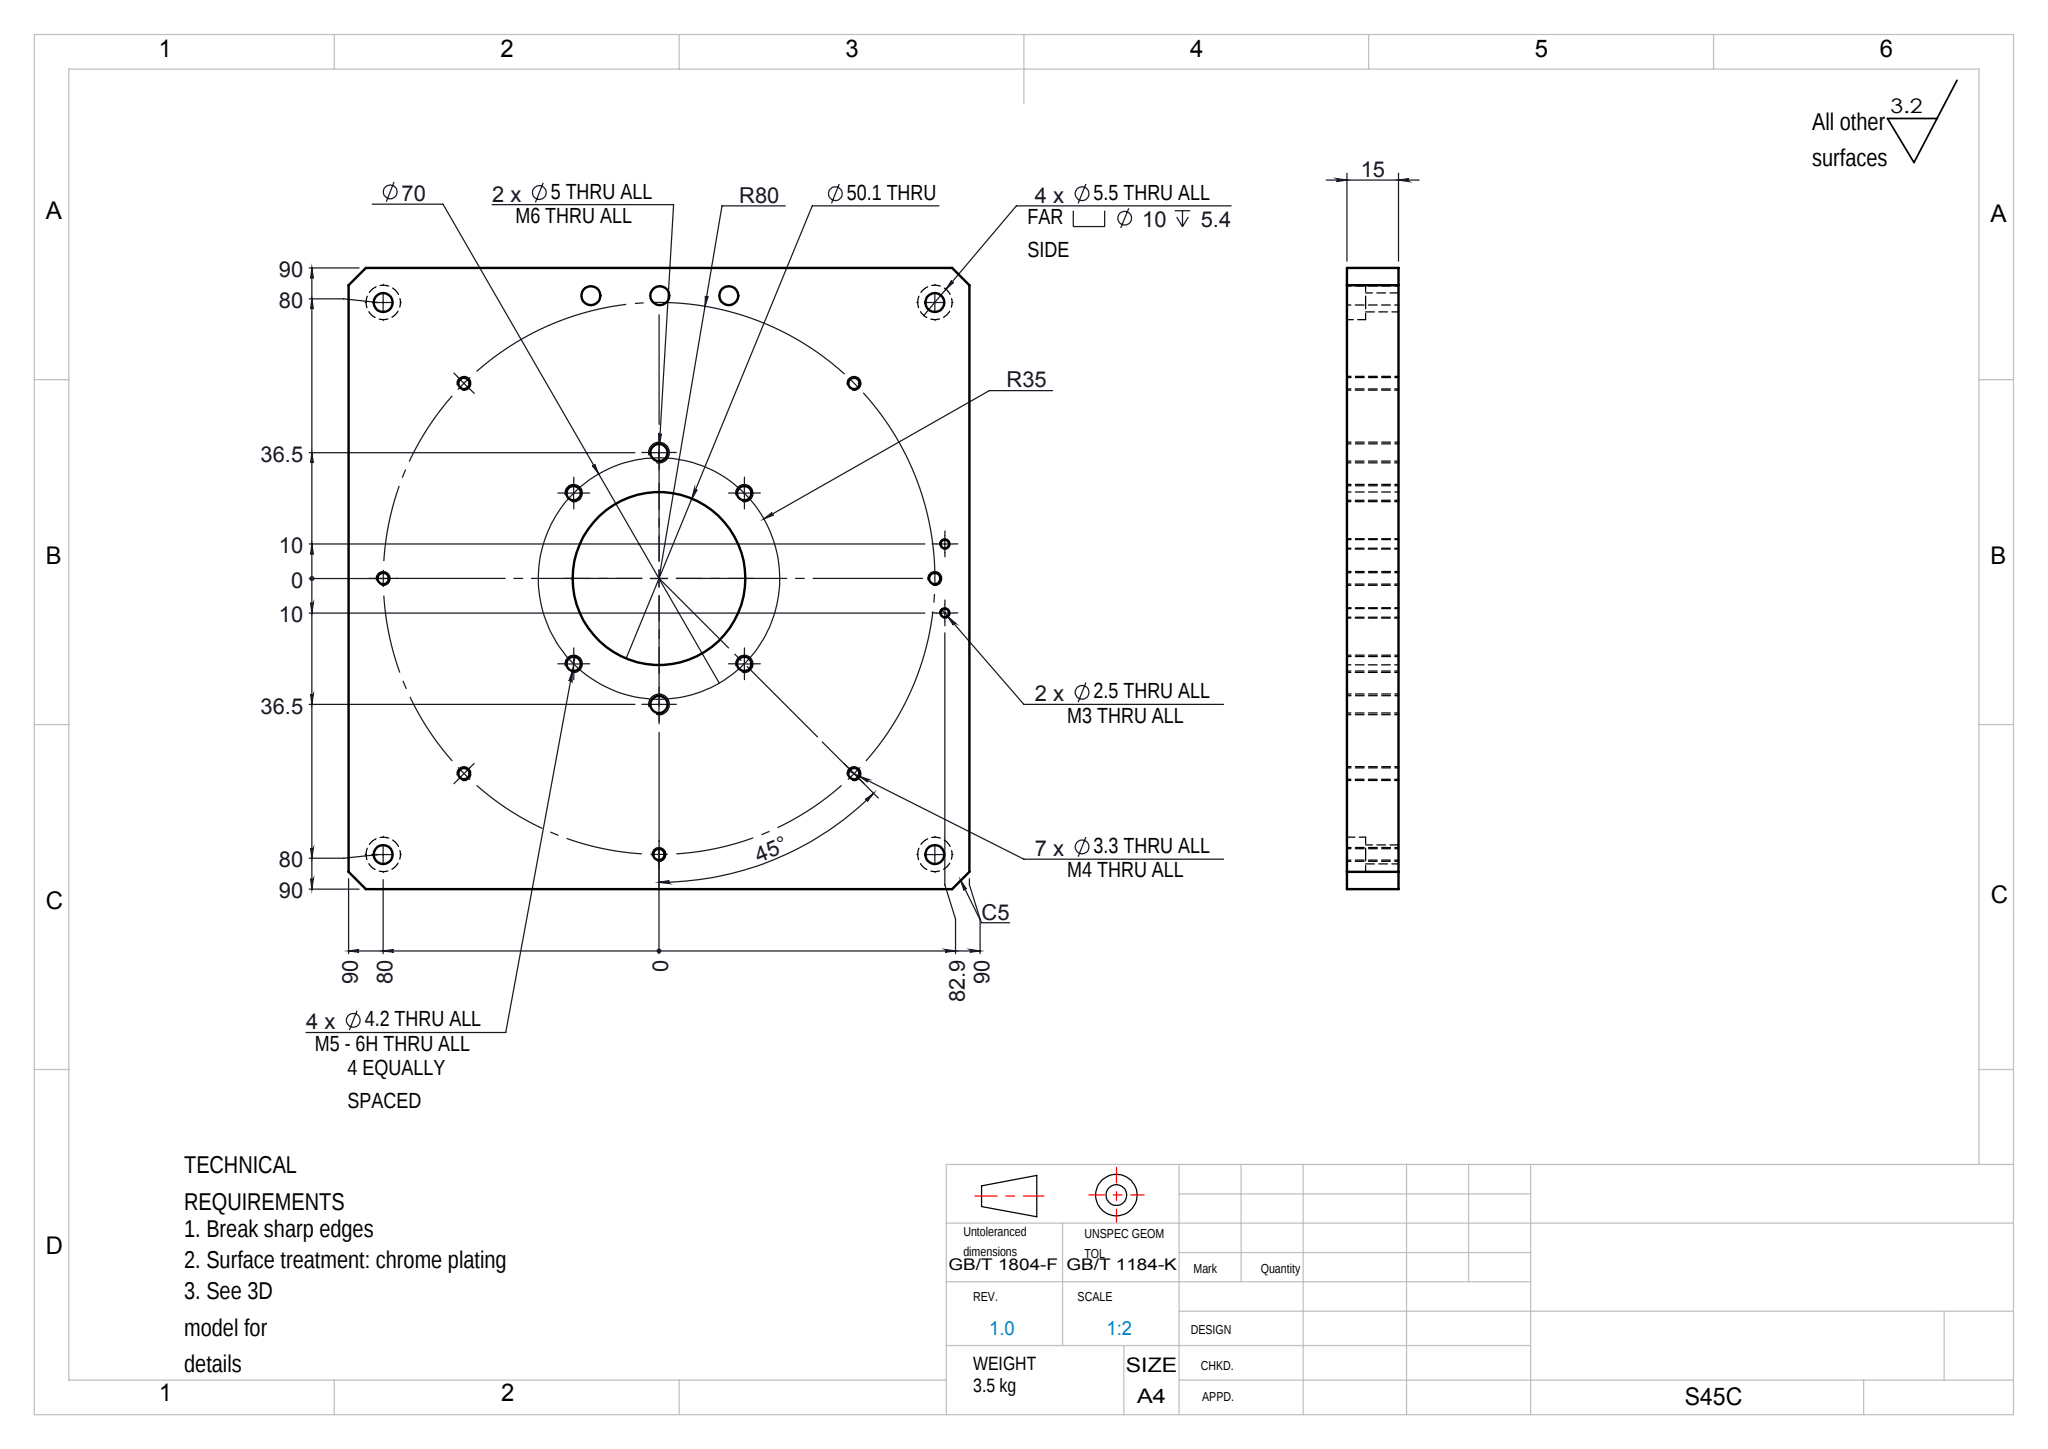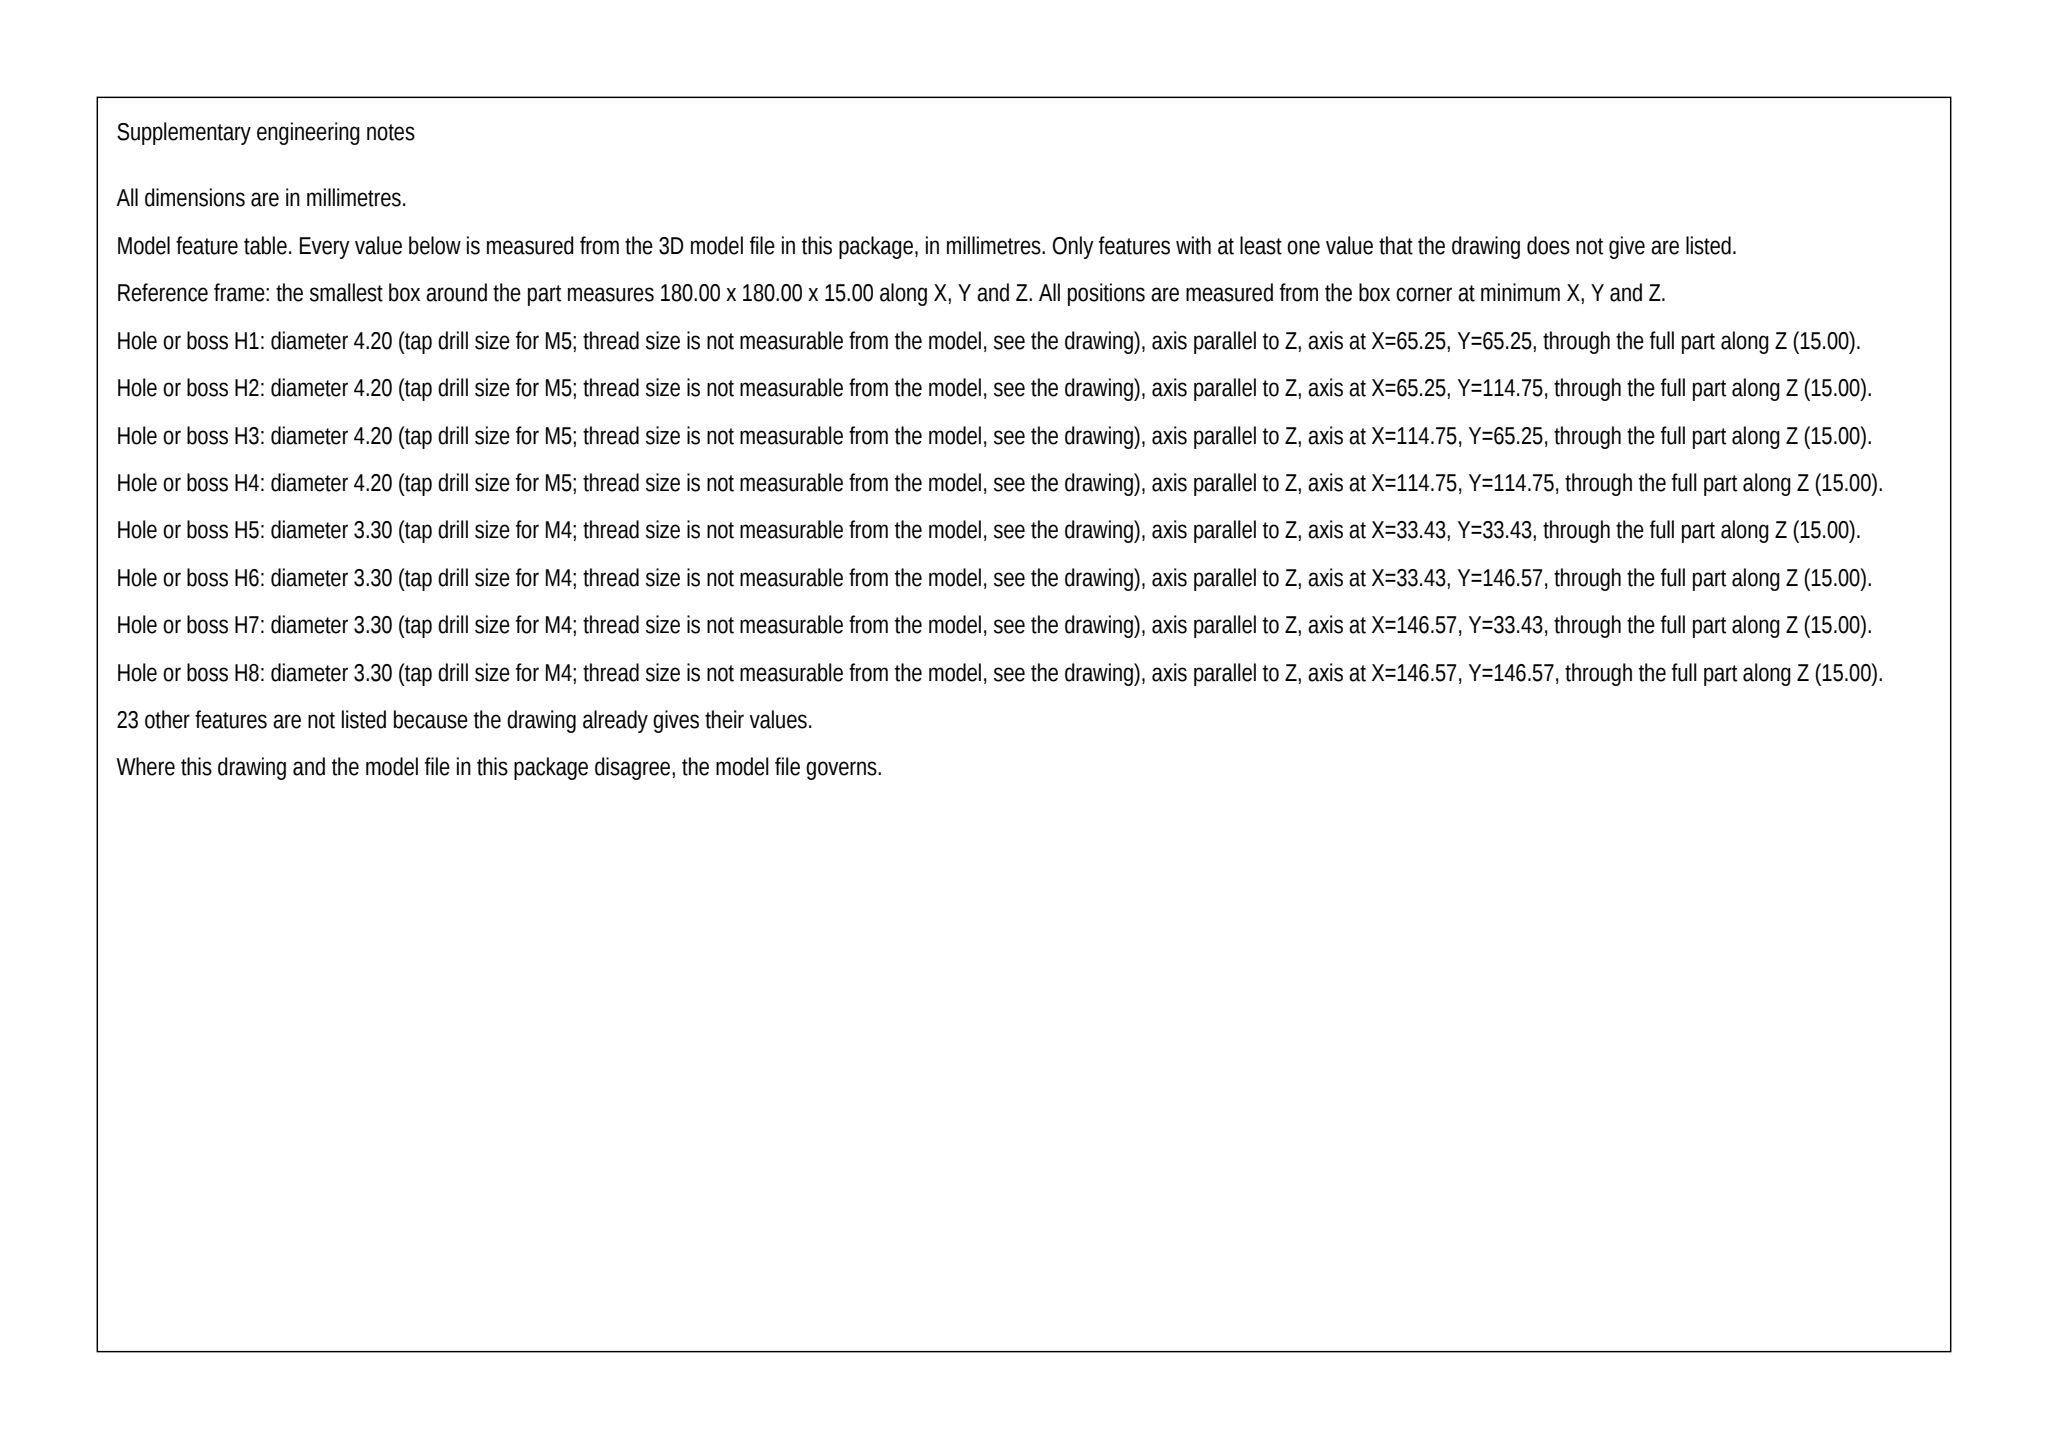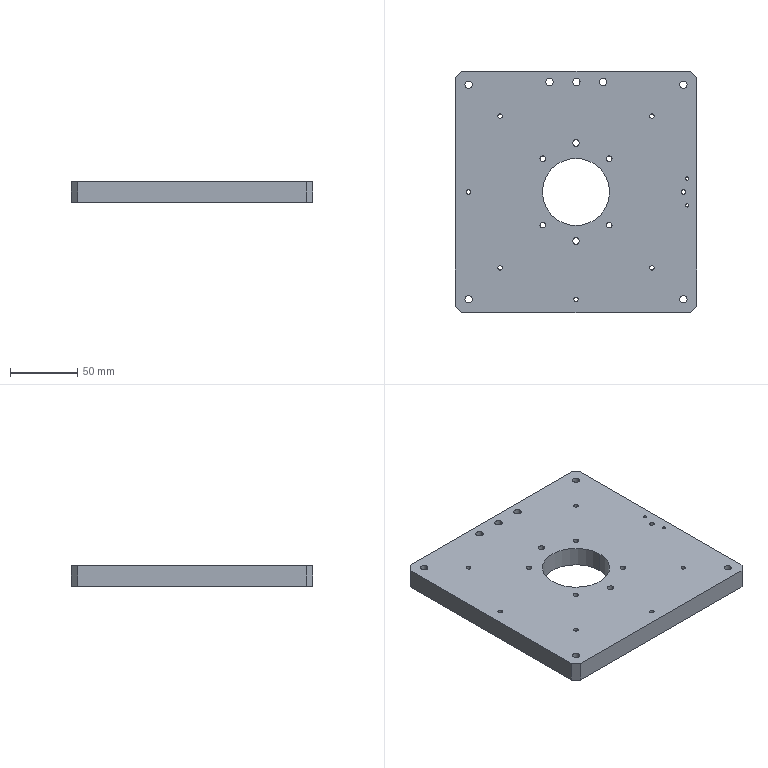Part | SolidWorks | mm | 1 solid | 68 faces | box 180 x 180 x 15 mm | volume 449536 mm3 | cylinder 54 | plane 14 | commonest cylinder face diameters 5.5 x14 3.3 x14 4.2 x8 10 x8 5 x4 2.5 x4 50.1 x2
build123d program:
from build123d import *

# Parameters (mm, degrees)
SKETCH1_W                                       = 180
SKETCH1_H                                       = 180
BOSS_EXTRUDE1_DEPTH                             = 15
M5_HEX_SOCKET_HEAD_CAP_SCREW_CBORE1_D           = 5.5
M5_HEX_SOCKET_HEAD_CAP_SCREW_CBORE1_CBORE_D     = 10
M5_HEX_SOCKET_HEAD_CAP_SCREW_CBORE1_CBORE_DEPTH = 5.4
SKETCH4_R                                       = 25.05
CUT_EXTRUDE1_DEPTH                              = 129.16
CHAMFER1_SIZE                                   = 5
M5_TAPPED_HOLE1_D                               = 4.2
M4_TAPPED_HOLE1_D                               = 3.3
M3_TAPPED_HOLE1_D                               = 2.5
M6_TAPPED_HOLE2_D                               = 5
M5_CLEARANCE_HOLE1_D                            = 5.5


with BuildPart() as part:
    # Sketch1 → Boss-Extrude1 (new body)
    with BuildSketch(Plane.XY):
        Rectangle(SKETCH1_W, SKETCH1_H)
    extrude(amount=BOSS_EXTRUDE1_DEPTH)

    # M5 Hex Socket Head Cap Screw CBORE1 (through all)
    with Locations(Plane(origin=(0, 0, 0), x_dir=(-1, 0, 0), z_dir=(0, 0, -1))):
        with Locations((-80, 80), (80, 80), (80, -80), (-80, -80)):
            CounterBoreHole(M5_HEX_SOCKET_HEAD_CAP_SCREW_CBORE1_D / 2, M5_HEX_SOCKET_HEAD_CAP_SCREW_CBORE1_CBORE_D / 2, M5_HEX_SOCKET_HEAD_CAP_SCREW_CBORE1_CBORE_DEPTH)

    # Sketch4 → Cut-Extrude1 (cut, through all)
    with BuildSketch(Plane(origin=(0, 0, 0), x_dir=(-1, 0, 0), z_dir=(0, 0, -1))):
        Circle(SKETCH4_R)
    extrude(amount=-CUT_EXTRUDE1_DEPTH, mode=Mode.SUBTRACT)

    # Chamfer1
    chamfer1_edges = [part.edges().sort_by_distance(p)[0] for p in [
        (90, -90, 7.5),
        (-90, -90, 7.5),
        (-90, 90, 7.5),
        (90, 90, 7.5),
    ]]
    chamfer(chamfer1_edges, length=CHAMFER1_SIZE)

    # M5 Tapped Hole1 (through all)
    with Locations(Plane.XY.offset(15)):
        with Locations((24.749, 24.749), (-24.749, 24.749), (-24.749, -24.749), (24.749, -24.749)):
            Hole(M5_TAPPED_HOLE1_D / 2)

    # M4 Tapped Hole1 (through all)
    with Locations(Plane.XY.offset(15)):
        with Locations((56.569, -56.569), (0, -80), (-56.569, -56.569), (-80, 0), (-56.569, 56.569), (80, 0), (56.569, 56.569)):
            Hole(M4_TAPPED_HOLE1_D / 2)

    # M3 Tapped Hole1 (through all)
    with Locations(Plane(origin=(0, 0, 0), x_dir=(1, 0, 0), z_dir=(0, 0, -1))):
        with Locations((82.9, 10), (82.9, -10)):
            Hole(M3_TAPPED_HOLE1_D / 2)

    # M6 Tapped Hole2 (through all)
    with Locations(Plane(origin=(0, 0, 0), x_dir=(-1, 0, 0), z_dir=(0, 0, -1))):
        with Locations((0, -36.5), (0, 36.5)):
            Hole(M6_TAPPED_HOLE2_D / 2)

    # M5 Clearance Hole1 (through all)
    with Locations(Plane.XY.offset(15)):
        with Locations((-19.75, 82), (0.25, 82), (20.25, 82)):
            Hole(M5_CLEARANCE_HOLE1_D / 2)


solid = part.part